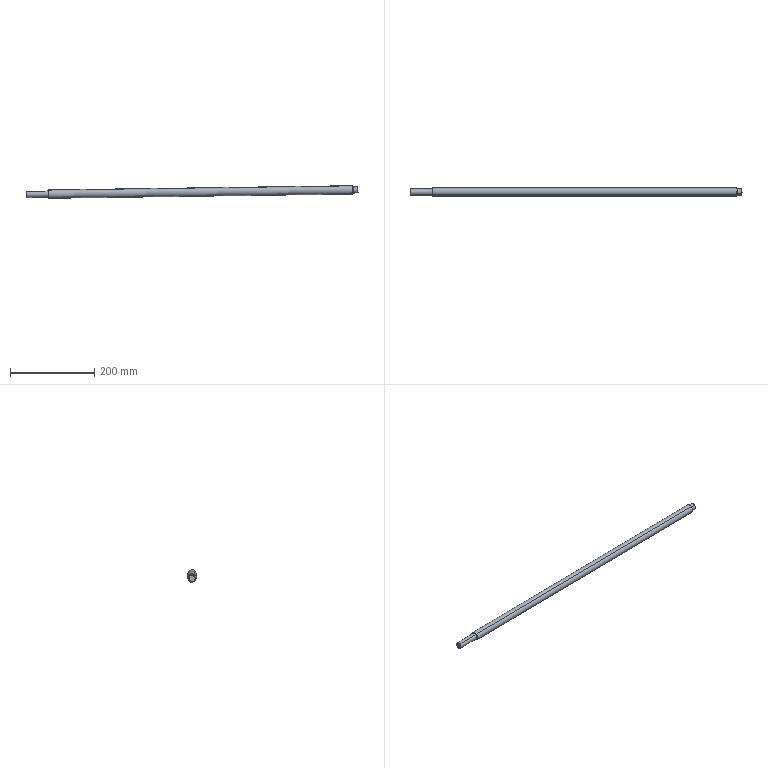Component | SolidWorks | DA-0220-Screw-4 | 1 solid | 18 faces | box 790.12 x 20.29 x 30.1 mm | volume 239115 mm3 | cylinder 6 | torus 4 | cone 4 | plane 4 | commonest cylinder face diameters 15 x4 20 x2
build123d program:
from build123d import *

# Parameters (mm, degrees)
CHAMFER1_SIZE = 0.3
FILLET1_R     = 0.5


with BuildPart() as part:
    # Sketch1 → Revolve1 (revolve)
    with BuildSketch(Plane.XY):
        Polygon((0, 7.49), (0, -0.01047), (790, -0.01047), (790, 7.49), (778, 7.49), (778, 9.99), (54, 9.99), (54, 7.49), align=None)
    revolve(axis=Axis((0, -0.01047, 0), (1, 0, 0)))

    # Chamfer1
    chamfer1_edges = [part.edges().sort_by_distance(p)[0] for p in [
        (0, -7.51, 0),
        (790, -7.51, 0),
    ]]
    chamfer(chamfer1_edges, length=CHAMFER1_SIZE)

    # Fillet1
    fillet1_edges = [part.edges().sort_by_distance(p)[0] for p in [
        (54, -7.51, 0),
        (778, -7.51, 0),
    ]]
    fillet(fillet1_edges, radius=FILLET1_R)


solid = part.part

# Placed as in the assembly
solid = solid.moved(Location((248.156, -93.945, 6.971), (44.973, -0.5493, 0.5815)))
STEP:
#1=COLOUR_RGB('',0.7922,0.8196,0.9333);
#2=FILL_AREA_STYLE_COLOUR('',#1);
#3=FILL_AREA_STYLE('',(#2));
#4=SURFACE_STYLE_FILL_AREA(#3);
#5=SURFACE_SIDE_STYLE('',(#4));
#6=SURFACE_STYLE_USAGE(.BOTH.,#5);
#7=PRESENTATION_STYLE_ASSIGNMENT((#6));
#8=CARTESIAN_POINT('',(40.413,-3.838,0.955));
#9=VERTEX_POINT('',#8);
#10=CARTESIAN_POINT('',(40.42,-3.535,0.4487));
#11=VERTEX_POINT('',#10);
#12=CARTESIAN_POINT('',(40.417,-3.687,0.7019));
#13=DIRECTION('',(0.9999,0.000404,0.01395));
#14=DIRECTION('',(0.01176,0.5145,-0.8574));
#15=AXIS2_PLACEMENT_3D('',#12,#13,#14);
#16=CIRCLE('',#15,0.2953);
#17=EDGE_CURVE('',#9,#11,#16,.T.);
#18=ORIENTED_EDGE('',*,*,#17,.F.);
#19=CARTESIAN_POINT('',(40.393,-3.849,0.9716));
#20=VERTEX_POINT('',#19);
#21=CARTESIAN_POINT('',(40.413,-3.849,0.9719));
#22=DIRECTION('',(-0.007525,0.8575,0.5144));
#23=DIRECTION('',(0.,-0.5144,0.8575));
#24=AXIS2_PLACEMENT_3D('',#21,#22,#23);
#25=CIRCLE('',#24,0.01969);
#26=EDGE_CURVE('',#9,#20,#25,.T.);
#27=ORIENTED_EDGE('',*,*,#26,.T.);
#28=CARTESIAN_POINT('',(40.401,-3.524,0.4315));
#29=VERTEX_POINT('',#28);
#30=CARTESIAN_POINT('',(40.397,-3.687,0.7016));
#31=DIRECTION('',(-0.9999,-0.000404,-0.01395));
#32=DIRECTION('',(0.01176,0.5145,-0.8574));
#33=AXIS2_PLACEMENT_3D('',#30,#31,#32);
#34=CIRCLE('',#33,0.315);
#35=EDGE_CURVE('',#29,#20,#34,.T.);
#36=ORIENTED_EDGE('',*,*,#35,.F.);
#37=CARTESIAN_POINT('',(40.42,-3.524,0.4318));
#38=DIRECTION('',(0.007525,-0.8575,-0.5144));
#39=DIRECTION('',(0.,0.5144,-0.8575));
#40=AXIS2_PLACEMENT_3D('',#37,#38,#39);
#41=CIRCLE('',#40,0.01969);
#42=EDGE_CURVE('',#11,#29,#41,.T.);
#43=ORIENTED_EDGE('',*,*,#42,.F.);
#44=EDGE_LOOP('',(#18,#27,#36,#43));
#45=FACE_OUTER_BOUND('',#44,.T.);
#46=CARTESIAN_POINT('',(40.417,-3.687,0.7019));
#47=DIRECTION('',(0.9999,0.000404,0.01395));
#48=DIRECTION('',(0.01176,0.5145,-0.8574));
#49=AXIS2_PLACEMENT_3D('',#46,#47,#48);
#50=TOROIDAL_SURFACE('',#49,0.315,0.01969);
#51=ADVANCED_FACE('',(#45),#50,.F.);
#52=CARTESIAN_POINT('',(11.879,-3.546,0.05038));
#53=VERTEX_POINT('',#52);
#54=CARTESIAN_POINT('',(11.873,-3.85,0.5567));
#55=VERTEX_POINT('',#54);
#56=CARTESIAN_POINT('',(11.876,-3.698,0.3036));
#57=DIRECTION('',(-0.9999,-0.000404,-0.01395));
#58=DIRECTION('',(-0.01176,-0.5145,0.8574));
#59=AXIS2_PLACEMENT_3D('',#56,#57,#58);
#60=CIRCLE('',#59,0.2953);
#61=EDGE_CURVE('',#53,#55,#60,.T.);
#62=ORIENTED_EDGE('',*,*,#61,.F.);
#63=CARTESIAN_POINT('',(11.899,-3.536,0.03378));
#64=VERTEX_POINT('',#63);
#65=CARTESIAN_POINT('',(11.88,-3.536,0.0335));
#66=DIRECTION('',(-0.007525,0.8575,0.5144));
#67=DIRECTION('',(0.,-0.5144,0.8575));
#68=AXIS2_PLACEMENT_3D('',#65,#66,#67);
#69=CIRCLE('',#68,0.01969);
#70=EDGE_CURVE('',#53,#64,#69,.T.);
#71=ORIENTED_EDGE('',*,*,#70,.T.);
#72=CARTESIAN_POINT('',(11.892,-3.86,0.5739));
#73=VERTEX_POINT('',#72);
#74=CARTESIAN_POINT('',(11.896,-3.698,0.3038));
#75=DIRECTION('',(0.9999,0.000404,0.01395));
#76=DIRECTION('',(-0.01176,-0.5145,0.8574));
#77=AXIS2_PLACEMENT_3D('',#74,#75,#76);
#78=CIRCLE('',#77,0.315);
#79=EDGE_CURVE('',#73,#64,#78,.T.);
#80=ORIENTED_EDGE('',*,*,#79,.F.);
#81=CARTESIAN_POINT('',(11.872,-3.86,0.5736));
#82=DIRECTION('',(0.007525,-0.8575,-0.5144));
#83=DIRECTION('',(0.,0.5144,-0.8575));
#84=AXIS2_PLACEMENT_3D('',#81,#82,#83);
#85=CIRCLE('',#84,0.01969);
#86=EDGE_CURVE('',#55,#73,#85,.T.);
#87=ORIENTED_EDGE('',*,*,#86,.F.);
#88=EDGE_LOOP('',(#62,#71,#80,#87));
#89=FACE_OUTER_BOUND('',#88,.T.);
#90=CARTESIAN_POINT('',(11.876,-3.698,0.3036));
#91=DIRECTION('',(-0.9999,-0.000404,-0.01395));
#92=DIRECTION('',(-0.01176,-0.5145,0.8574));
#93=AXIS2_PLACEMENT_3D('',#90,#91,#92);
#94=TOROIDAL_SURFACE('',#93,0.315,0.01969);
#95=ADVANCED_FACE('',(#89),#94,.F.);
#96=CARTESIAN_POINT('',(40.871,-3.929,0.5624));
#97=VERTEX_POINT('',#96);
#98=CARTESIAN_POINT('',(40.867,-3.443,0.854));
#99=VERTEX_POINT('',#98);
#100=CARTESIAN_POINT('',(40.869,-3.686,0.7082));
#101=DIRECTION('',(0.9999,0.000404,0.01395));
#102=DIRECTION('',(0.01176,0.5145,-0.8574));
#103=AXIS2_PLACEMENT_3D('',#100,#101,#102);
#104=CIRCLE('',#103,0.2835);
#105=EDGE_CURVE('',#97,#99,#104,.T.);
#106=ORIENTED_EDGE('',*,*,#105,.F.);
#107=CARTESIAN_POINT('',(40.86,-3.94,0.5561));
#108=VERTEX_POINT('',#107);
#109=CARTESIAN_POINT('',(40.871,-3.929,0.5624));
#110=DIRECTION('',(-0.7017,-0.6066,-0.3736));
#111=VECTOR('',#110,39.37);
#112=LINE('',#109,#111);
#113=EDGE_CURVE('',#97,#108,#112,.T.);
#114=ORIENTED_EDGE('',*,*,#113,.T.);
#115=CARTESIAN_POINT('',(40.861,-3.534,0.4548));
#116=VERTEX_POINT('',#115);
#117=CARTESIAN_POINT('',(40.857,-3.686,0.708));
#118=DIRECTION('',(-0.9999,-0.000404,-0.01395));
#119=DIRECTION('',(0.007525,-0.8575,-0.5144));
#120=AXIS2_PLACEMENT_3D('',#117,#118,#119);
#121=CIRCLE('',#120,0.2953);
#122=EDGE_CURVE('',#116,#108,#121,.T.);
#123=ORIENTED_EDGE('',*,*,#122,.F.);
#124=CARTESIAN_POINT('',(40.855,-3.433,0.8599));
#125=VERTEX_POINT('',#124);
#126=CARTESIAN_POINT('',(40.857,-3.686,0.708));
#127=DIRECTION('',(-0.9999,-0.000404,-0.01395));
#128=DIRECTION('',(0.007525,-0.8575,-0.5144));
#129=AXIS2_PLACEMENT_3D('',#126,#127,#128);
#130=CIRCLE('',#129,0.2953);
#131=EDGE_CURVE('',#125,#116,#130,.T.);
#132=ORIENTED_EDGE('',*,*,#131,.F.);
#133=CARTESIAN_POINT('',(40.867,-3.443,0.854));
#134=DIRECTION('',(-0.7124,0.6061,0.3539));
#135=VECTOR('',#134,39.37);
#136=LINE('',#133,#135);
#137=EDGE_CURVE('',#99,#125,#136,.T.);
#138=ORIENTED_EDGE('',*,*,#137,.F.);
#139=EDGE_LOOP('',(#106,#114,#123,#132,#138));
#140=FACE_OUTER_BOUND('',#139,.T.);
#141=CARTESIAN_POINT('',(40.869,-3.686,0.7082));
#142=DIRECTION('',(-0.9999,-0.000404,-0.01395));
#143=DIRECTION('',(-0.007525,0.8575,0.5144));
#144=AXIS2_PLACEMENT_3D('',#141,#142,#143);
#145=CONICAL_SURFACE('',#144,0.2835,0.7854);
#146=ADVANCED_FACE('',(#140),#145,.T.);
#147=CARTESIAN_POINT('',(9.768,-3.456,0.42));
#148=VERTEX_POINT('',#147);
#149=CARTESIAN_POINT('',(9.772,-3.942,0.1283));
#150=VERTEX_POINT('',#149);
#151=CARTESIAN_POINT('',(9.77,-3.699,0.2742));
#152=DIRECTION('',(-0.9999,-0.000404,-0.01395));
#153=DIRECTION('',(-0.01176,-0.5145,0.8574));
#154=AXIS2_PLACEMENT_3D('',#151,#152,#153);
#155=CIRCLE('',#154,0.2835);
#156=EDGE_CURVE('',#148,#150,#155,.T.);
#157=ORIENTED_EDGE('',*,*,#156,.F.);
#158=CARTESIAN_POINT('',(9.78,-3.446,0.4262));
#159=VERTEX_POINT('',#158);
#160=CARTESIAN_POINT('',(9.78,-3.446,0.4262));
#161=DIRECTION('',(0.7017,0.6066,0.3736));
#162=VECTOR('',#161,39.37);
#163=LINE('',#160,#162);
#164=EDGE_CURVE('',#148,#159,#163,.T.);
#165=ORIENTED_EDGE('',*,*,#164,.T.);
#166=CARTESIAN_POINT('',(9.785,-3.547,0.02115));
#167=VERTEX_POINT('',#166);
#168=CARTESIAN_POINT('',(9.782,-3.699,0.2743));
#169=DIRECTION('',(0.9999,0.000404,0.01395));
#170=DIRECTION('',(-0.007525,0.8575,0.5144));
#171=AXIS2_PLACEMENT_3D('',#168,#169,#170);
#172=CIRCLE('',#171,0.2953);
#173=EDGE_CURVE('',#167,#159,#172,.T.);
#174=ORIENTED_EDGE('',*,*,#173,.F.);
#175=CARTESIAN_POINT('',(9.784,-3.952,0.1224));
#176=VERTEX_POINT('',#175);
#177=CARTESIAN_POINT('',(9.782,-3.699,0.2743));
#178=DIRECTION('',(0.9999,0.000404,0.01395));
#179=DIRECTION('',(-0.007525,0.8575,0.5144));
#180=AXIS2_PLACEMENT_3D('',#177,#178,#179);
#181=CIRCLE('',#180,0.2953);
#182=EDGE_CURVE('',#176,#167,#181,.T.);
#183=ORIENTED_EDGE('',*,*,#182,.F.);
#184=CARTESIAN_POINT('',(9.784,-3.952,0.1224));
#185=DIRECTION('',(0.7124,-0.6061,-0.3539));
#186=VECTOR('',#185,39.37);
#187=LINE('',#184,#186);
#188=EDGE_CURVE('',#150,#176,#187,.T.);
#189=ORIENTED_EDGE('',*,*,#188,.F.);
#190=EDGE_LOOP('',(#157,#165,#174,#183,#189));
#191=FACE_OUTER_BOUND('',#190,.T.);
#192=CARTESIAN_POINT('',(9.782,-3.699,0.2743));
#193=DIRECTION('',(0.9999,0.000404,0.01395));
#194=DIRECTION('',(0.007525,-0.8575,-0.5144));
#195=AXIS2_PLACEMENT_3D('',#192,#193,#194);
#196=CONICAL_SURFACE('',#195,0.2953,0.7854);
#197=ADVANCED_FACE('',(#191),#196,.T.);
#198=ORIENTED_EDGE('',*,*,#173,.T.);
#199=CARTESIAN_POINT('',(9.778,-3.851,0.5275));
#200=VERTEX_POINT('',#199);
#201=CARTESIAN_POINT('',(9.782,-3.699,0.2743));
#202=DIRECTION('',(0.9999,0.000404,0.01395));
#203=DIRECTION('',(-0.007525,0.8575,0.5144));
#204=AXIS2_PLACEMENT_3D('',#201,#202,#203);
#205=CIRCLE('',#204,0.2953);
#206=EDGE_CURVE('',#159,#200,#205,.T.);
#207=ORIENTED_EDGE('',*,*,#206,.T.);
#208=CARTESIAN_POINT('',(9.766,-3.851,0.5273));
#209=DIRECTION('',(0.9999,0.000404,0.01395));
#210=VECTOR('',#209,39.37);
#211=LINE('',#208,#210);
#212=EDGE_CURVE('',#200,#55,#211,.T.);
#213=ORIENTED_EDGE('',*,*,#212,.T.);
#214=CARTESIAN_POINT('',(11.876,-3.698,0.3036));
#215=DIRECTION('',(-0.9999,-0.000404,-0.01395));
#216=DIRECTION('',(-0.01176,-0.5145,0.8574));
#217=AXIS2_PLACEMENT_3D('',#214,#215,#216);
#218=CIRCLE('',#217,0.2953);
#219=EDGE_CURVE('',#55,#53,#218,.T.);
#220=ORIENTED_EDGE('',*,*,#219,.T.);
#221=CARTESIAN_POINT('',(9.773,-3.547,0.02099));
#222=DIRECTION('',(0.9999,0.000404,0.01395));
#223=VECTOR('',#222,39.37);
#224=LINE('',#221,#223);
#225=EDGE_CURVE('',#167,#53,#224,.T.);
#226=ORIENTED_EDGE('',*,*,#225,.F.);
#227=EDGE_LOOP('',(#198,#207,#213,#220,#226));
#228=FACE_OUTER_BOUND('',#227,.T.);
#229=CARTESIAN_POINT('',(9.77,-3.699,0.2742));
#230=DIRECTION('',(0.9999,0.000404,0.01395));
#231=DIRECTION('',(0.01176,0.5145,-0.8574));
#232=AXIS2_PLACEMENT_3D('',#229,#230,#231);
#233=CYLINDRICAL_SURFACE('',#232,0.2953);
#234=ADVANCED_FACE('',(#228),#233,.T.);
#235=CARTESIAN_POINT('',(11.9,-3.495,-0.03374));
#236=VERTEX_POINT('',#235);
#237=CARTESIAN_POINT('',(11.891,-3.901,0.6414));
#238=VERTEX_POINT('',#237);
#239=CARTESIAN_POINT('',(11.896,-3.698,0.3038));
#240=DIRECTION('',(0.9999,0.000404,0.01395));
#241=DIRECTION('',(0.01176,0.5145,-0.8574));
#242=AXIS2_PLACEMENT_3D('',#239,#240,#241);
#243=CIRCLE('',#242,0.3937);
#244=EDGE_CURVE('',#236,#238,#243,.T.);
#245=ORIENTED_EDGE('',*,*,#244,.T.);
#246=CARTESIAN_POINT('',(40.392,-3.889,1.039));
#247=VERTEX_POINT('',#246);
#248=CARTESIAN_POINT('',(9.765,-3.901,0.6117));
#249=DIRECTION('',(0.9999,0.000404,0.01395));
#250=VECTOR('',#249,39.37);
#251=LINE('',#248,#250);
#252=EDGE_CURVE('',#238,#247,#251,.T.);
#253=ORIENTED_EDGE('',*,*,#252,.T.);
#254=CARTESIAN_POINT('',(40.401,-3.484,0.364));
#255=VERTEX_POINT('',#254);
#256=CARTESIAN_POINT('',(40.397,-3.687,0.7016));
#257=DIRECTION('',(0.9999,0.000404,0.01395));
#258=DIRECTION('',(0.01176,0.5145,-0.8574));
#259=AXIS2_PLACEMENT_3D('',#256,#257,#258);
#260=CIRCLE('',#259,0.3937);
#261=EDGE_CURVE('',#255,#247,#260,.T.);
#262=ORIENTED_EDGE('',*,*,#261,.F.);
#263=CARTESIAN_POINT('',(9.775,-3.496,-0.0634));
#264=DIRECTION('',(0.9999,0.000404,0.01395));
#265=VECTOR('',#264,39.37);
#266=LINE('',#263,#265);
#267=EDGE_CURVE('',#236,#255,#266,.T.);
#268=ORIENTED_EDGE('',*,*,#267,.F.);
#269=EDGE_LOOP('',(#245,#253,#262,#268));
#270=FACE_OUTER_BOUND('',#269,.T.);
#271=CARTESIAN_POINT('',(9.77,-3.699,0.2742));
#272=DIRECTION('',(0.9999,0.000404,0.01395));
#273=DIRECTION('',(0.01176,0.5145,-0.8574));
#274=AXIS2_PLACEMENT_3D('',#271,#272,#273);
#275=CYLINDRICAL_SURFACE('',#274,0.3937);
#276=ADVANCED_FACE('',(#270),#275,.T.);
#277=CARTESIAN_POINT('',(40.417,-3.687,0.7019));
#278=DIRECTION('',(0.9999,0.000404,0.01395));
#279=DIRECTION('',(0.01176,0.5145,-0.8574));
#280=AXIS2_PLACEMENT_3D('',#277,#278,#279);
#281=CIRCLE('',#280,0.2953);
#282=EDGE_CURVE('',#11,#9,#281,.T.);
#283=ORIENTED_EDGE('',*,*,#282,.T.);
#284=CARTESIAN_POINT('',(40.854,-3.838,0.9612));
#285=VERTEX_POINT('',#284);
#286=CARTESIAN_POINT('',(9.766,-3.851,0.5273));
#287=DIRECTION('',(0.9999,0.000404,0.01395));
#288=VECTOR('',#287,39.37);
#289=LINE('',#286,#288);
#290=EDGE_CURVE('',#9,#285,#289,.T.);
#291=ORIENTED_EDGE('',*,*,#290,.T.);
#292=CARTESIAN_POINT('',(40.857,-3.686,0.708));
#293=DIRECTION('',(-0.9999,-0.000404,-0.01395));
#294=DIRECTION('',(0.007525,-0.8575,-0.5144));
#295=AXIS2_PLACEMENT_3D('',#292,#293,#294);
#296=CIRCLE('',#295,0.2953);
#297=EDGE_CURVE('',#285,#125,#296,.T.);
#298=ORIENTED_EDGE('',*,*,#297,.T.);
#299=ORIENTED_EDGE('',*,*,#131,.T.);
#300=CARTESIAN_POINT('',(9.773,-3.547,0.02099));
#301=DIRECTION('',(0.9999,0.000404,0.01395));
#302=VECTOR('',#301,39.37);
#303=LINE('',#300,#302);
#304=EDGE_CURVE('',#11,#116,#303,.T.);
#305=ORIENTED_EDGE('',*,*,#304,.F.);
#306=EDGE_LOOP('',(#283,#291,#298,#299,#305));
#307=FACE_OUTER_BOUND('',#306,.T.);
#308=CARTESIAN_POINT('',(9.77,-3.699,0.2742));
#309=DIRECTION('',(0.9999,0.000404,0.01395));
#310=DIRECTION('',(0.01176,0.5145,-0.8574));
#311=AXIS2_PLACEMENT_3D('',#308,#309,#310);
#312=CYLINDRICAL_SURFACE('',#311,0.2953);
#313=ADVANCED_FACE('',(#307),#312,.T.);
#314=CARTESIAN_POINT('',(40.869,-3.686,0.7082));
#315=DIRECTION('',(0.9999,0.000404,0.01395));
#316=DIRECTION('',(0.01176,0.5145,-0.8574));
#317=AXIS2_PLACEMENT_3D('',#314,#315,#316);
#318=CIRCLE('',#317,0.2835);
#319=EDGE_CURVE('',#99,#97,#318,.T.);
#320=ORIENTED_EDGE('',*,*,#319,.T.);
#321=ORIENTED_EDGE('',*,*,#105,.T.);
#322=EDGE_LOOP('',(#320,#321));
#323=FACE_OUTER_BOUND('',#322,.T.);
#324=CARTESIAN_POINT('',(40.869,-3.686,0.7082));
#325=DIRECTION('',(0.9999,0.000404,0.01395));
#326=DIRECTION('',(0.01176,0.5145,-0.8574));
#327=AXIS2_PLACEMENT_3D('',#324,#325,#326);
#328=PLANE('',#327);
#329=ADVANCED_FACE('',(#323),#328,.T.);
#330=ORIENTED_EDGE('',*,*,#290,.F.);
#331=ORIENTED_EDGE('',*,*,#17,.T.);
#332=ORIENTED_EDGE('',*,*,#304,.T.);
#333=ORIENTED_EDGE('',*,*,#122,.T.);
#334=CARTESIAN_POINT('',(40.857,-3.686,0.708));
#335=DIRECTION('',(-0.9999,-0.000404,-0.01395));
#336=DIRECTION('',(0.007525,-0.8575,-0.5144));
#337=AXIS2_PLACEMENT_3D('',#334,#335,#336);
#338=CIRCLE('',#337,0.2953);
#339=EDGE_CURVE('',#108,#285,#338,.T.);
#340=ORIENTED_EDGE('',*,*,#339,.T.);
#341=EDGE_LOOP('',(#330,#331,#332,#333,#340));
#342=FACE_OUTER_BOUND('',#341,.T.);
#343=CARTESIAN_POINT('',(9.77,-3.699,0.2742));
#344=DIRECTION('',(0.9999,0.000404,0.01395));
#345=DIRECTION('',(0.01176,0.5145,-0.8574));
#346=AXIS2_PLACEMENT_3D('',#343,#344,#345);
#347=CYLINDRICAL_SURFACE('',#346,0.2953);
#348=ADVANCED_FACE('',(#342),#347,.T.);
#349=ORIENTED_EDGE('',*,*,#35,.T.);
#350=CARTESIAN_POINT('',(40.397,-3.687,0.7016));
#351=DIRECTION('',(-0.9999,-0.000404,-0.01395));
#352=DIRECTION('',(0.01176,0.5145,-0.8574));
#353=AXIS2_PLACEMENT_3D('',#350,#351,#352);
#354=CIRCLE('',#353,0.315);
#355=EDGE_CURVE('',#20,#29,#354,.T.);
#356=ORIENTED_EDGE('',*,*,#355,.T.);
#357=EDGE_LOOP('',(#349,#356));
#358=FACE_BOUND('',#357,.T.);
#359=ORIENTED_EDGE('',*,*,#261,.T.);
#360=CARTESIAN_POINT('',(40.397,-3.687,0.7016));
#361=DIRECTION('',(0.9999,0.000404,0.01395));
#362=DIRECTION('',(0.01176,0.5145,-0.8574));
#363=AXIS2_PLACEMENT_3D('',#360,#361,#362);
#364=CIRCLE('',#363,0.3937);
#365=EDGE_CURVE('',#247,#255,#364,.T.);
#366=ORIENTED_EDGE('',*,*,#365,.T.);
#367=EDGE_LOOP('',(#359,#366));
#368=FACE_OUTER_BOUND('',#367,.T.);
#369=CARTESIAN_POINT('',(40.4,-3.535,0.4484));
#370=DIRECTION('',(0.9999,0.000404,0.01395));
#371=DIRECTION('',(0.01176,0.5145,-0.8574));
#372=AXIS2_PLACEMENT_3D('',#369,#370,#371);
#373=PLANE('',#372);
#374=ADVANCED_FACE('',(#358,#368),#373,.T.);
#375=ORIENTED_EDGE('',*,*,#252,.F.);
#376=CARTESIAN_POINT('',(11.896,-3.698,0.3038));
#377=DIRECTION('',(0.9999,0.000404,0.01395));
#378=DIRECTION('',(0.01176,0.5145,-0.8574));
#379=AXIS2_PLACEMENT_3D('',#376,#377,#378);
#380=CIRCLE('',#379,0.3937);
#381=EDGE_CURVE('',#238,#236,#380,.T.);
#382=ORIENTED_EDGE('',*,*,#381,.T.);
#383=ORIENTED_EDGE('',*,*,#267,.T.);
#384=ORIENTED_EDGE('',*,*,#365,.F.);
#385=EDGE_LOOP('',(#375,#382,#383,#384));
#386=FACE_OUTER_BOUND('',#385,.T.);
#387=CARTESIAN_POINT('',(9.77,-3.699,0.2742));
#388=DIRECTION('',(0.9999,0.000404,0.01395));
#389=DIRECTION('',(0.01176,0.5145,-0.8574));
#390=AXIS2_PLACEMENT_3D('',#387,#388,#389);
#391=CYLINDRICAL_SURFACE('',#390,0.3937);
#392=ADVANCED_FACE('',(#386),#391,.T.);
#393=ORIENTED_EDGE('',*,*,#79,.T.);
#394=CARTESIAN_POINT('',(11.896,-3.698,0.3038));
#395=DIRECTION('',(0.9999,0.000404,0.01395));
#396=DIRECTION('',(-0.01176,-0.5145,0.8574));
#397=AXIS2_PLACEMENT_3D('',#394,#395,#396);
#398=CIRCLE('',#397,0.315);
#399=EDGE_CURVE('',#64,#73,#398,.T.);
#400=ORIENTED_EDGE('',*,*,#399,.T.);
#401=EDGE_LOOP('',(#393,#400));
#402=FACE_BOUND('',#401,.T.);
#403=ORIENTED_EDGE('',*,*,#244,.F.);
#404=ORIENTED_EDGE('',*,*,#381,.F.);
#405=EDGE_LOOP('',(#403,#404));
#406=FACE_OUTER_BOUND('',#405,.T.);
#407=CARTESIAN_POINT('',(11.9,-3.495,-0.03374));
#408=DIRECTION('',(-0.9999,-0.000404,-0.01395));
#409=DIRECTION('',(-0.01176,-0.5145,0.8574));
#410=AXIS2_PLACEMENT_3D('',#407,#408,#409);
#411=PLANE('',#410);
#412=ADVANCED_FACE('',(#402,#406),#411,.T.);
#413=ORIENTED_EDGE('',*,*,#212,.F.);
#414=CARTESIAN_POINT('',(9.782,-3.699,0.2743));
#415=DIRECTION('',(0.9999,0.000404,0.01395));
#416=DIRECTION('',(-0.007525,0.8575,0.5144));
#417=AXIS2_PLACEMENT_3D('',#414,#415,#416);
#418=CIRCLE('',#417,0.2953);
#419=EDGE_CURVE('',#200,#176,#418,.T.);
#420=ORIENTED_EDGE('',*,*,#419,.T.);
#421=ORIENTED_EDGE('',*,*,#182,.T.);
#422=ORIENTED_EDGE('',*,*,#225,.T.);
#423=ORIENTED_EDGE('',*,*,#61,.T.);
#424=EDGE_LOOP('',(#413,#420,#421,#422,#423));
#425=FACE_OUTER_BOUND('',#424,.T.);
#426=CARTESIAN_POINT('',(9.77,-3.699,0.2742));
#427=DIRECTION('',(0.9999,0.000404,0.01395));
#428=DIRECTION('',(0.01176,0.5145,-0.8574));
#429=AXIS2_PLACEMENT_3D('',#426,#427,#428);
#430=CYLINDRICAL_SURFACE('',#429,0.2953);
#431=ADVANCED_FACE('',(#425),#430,.T.);
#432=CARTESIAN_POINT('',(9.77,-3.699,0.2742));
#433=DIRECTION('',(-0.9999,-0.000404,-0.01395));
#434=DIRECTION('',(-0.01176,-0.5145,0.8574));
#435=AXIS2_PLACEMENT_3D('',#432,#433,#434);
#436=CIRCLE('',#435,0.2835);
#437=EDGE_CURVE('',#150,#148,#436,.T.);
#438=ORIENTED_EDGE('',*,*,#437,.T.);
#439=ORIENTED_EDGE('',*,*,#156,.T.);
#440=EDGE_LOOP('',(#438,#439));
#441=FACE_OUTER_BOUND('',#440,.T.);
#442=CARTESIAN_POINT('',(9.773,-3.547,0.02099));
#443=DIRECTION('',(-0.9999,-0.000404,-0.01395));
#444=DIRECTION('',(-0.01176,-0.5145,0.8574));
#445=AXIS2_PLACEMENT_3D('',#442,#443,#444);
#446=PLANE('',#445);
#447=ADVANCED_FACE('',(#441),#446,.T.);
#448=ORIENTED_EDGE('',*,*,#164,.F.);
#449=ORIENTED_EDGE('',*,*,#437,.F.);
#450=ORIENTED_EDGE('',*,*,#188,.T.);
#451=ORIENTED_EDGE('',*,*,#419,.F.);
#452=ORIENTED_EDGE('',*,*,#206,.F.);
#453=EDGE_LOOP('',(#448,#449,#450,#451,#452));
#454=FACE_OUTER_BOUND('',#453,.T.);
#455=CARTESIAN_POINT('',(9.782,-3.699,0.2743));
#456=DIRECTION('',(0.9999,0.000404,0.01395));
#457=DIRECTION('',(0.007525,-0.8575,-0.5144));
#458=AXIS2_PLACEMENT_3D('',#455,#456,#457);
#459=CONICAL_SURFACE('',#458,0.2953,0.7854);
#460=ADVANCED_FACE('',(#454),#459,.T.);
#461=ORIENTED_EDGE('',*,*,#113,.F.);
#462=ORIENTED_EDGE('',*,*,#319,.F.);
#463=ORIENTED_EDGE('',*,*,#137,.T.);
#464=ORIENTED_EDGE('',*,*,#297,.F.);
#465=ORIENTED_EDGE('',*,*,#339,.F.);
#466=EDGE_LOOP('',(#461,#462,#463,#464,#465));
#467=FACE_OUTER_BOUND('',#466,.T.);
#468=CARTESIAN_POINT('',(40.869,-3.686,0.7082));
#469=DIRECTION('',(-0.9999,-0.000404,-0.01395));
#470=DIRECTION('',(-0.007525,0.8575,0.5144));
#471=AXIS2_PLACEMENT_3D('',#468,#469,#470);
#472=CONICAL_SURFACE('',#471,0.2835,0.7854);
#473=ADVANCED_FACE('',(#467),#472,.T.);
#474=ORIENTED_EDGE('',*,*,#70,.F.);
#475=ORIENTED_EDGE('',*,*,#219,.F.);
#476=ORIENTED_EDGE('',*,*,#86,.T.);
#477=ORIENTED_EDGE('',*,*,#399,.F.);
#478=EDGE_LOOP('',(#474,#475,#476,#477));
#479=FACE_OUTER_BOUND('',#478,.T.);
#480=CARTESIAN_POINT('',(11.876,-3.698,0.3036));
#481=DIRECTION('',(-0.9999,-0.000404,-0.01395));
#482=DIRECTION('',(-0.01176,-0.5145,0.8574));
#483=AXIS2_PLACEMENT_3D('',#480,#481,#482);
#484=TOROIDAL_SURFACE('',#483,0.315,0.01969);
#485=ADVANCED_FACE('',(#479),#484,.F.);
#486=ORIENTED_EDGE('',*,*,#26,.F.);
#487=ORIENTED_EDGE('',*,*,#282,.F.);
#488=ORIENTED_EDGE('',*,*,#42,.T.);
#489=ORIENTED_EDGE('',*,*,#355,.F.);
#490=EDGE_LOOP('',(#486,#487,#488,#489));
#491=FACE_OUTER_BOUND('',#490,.T.);
#492=CARTESIAN_POINT('',(40.417,-3.687,0.7019));
#493=DIRECTION('',(0.9999,0.000404,0.01395));
#494=DIRECTION('',(0.01176,0.5145,-0.8574));
#495=AXIS2_PLACEMENT_3D('',#492,#493,#494);
#496=TOROIDAL_SURFACE('',#495,0.315,0.01969);
#497=ADVANCED_FACE('',(#491),#496,.F.);
#498=CLOSED_SHELL('',(#51,#95,#146,#197,#234,#276,#313,#329,#348,#374,#392,#412,#431,#447,#460,#473,#485,#497));
#499=MANIFOLD_SOLID_BREP('',#498);
#500=STYLED_ITEM('',(#7),#499);
#501=(LENGTH_UNIT()NAMED_UNIT(*)SI_UNIT($,.METRE.));
#502=LENGTH_MEASURE_WITH_UNIT(LENGTH_MEASURE(0.0254),#501);
#503=DIMENSIONAL_EXPONENTS(1.,0.,0.,0.,0.,0.,0.);
#504=(CONVERSION_BASED_UNIT('',#502)LENGTH_UNIT()NAMED_UNIT(#503));
#505=UNCERTAINTY_MEASURE_WITH_UNIT(LENGTH_MEASURE(0.00001),#504,'','');
#506=(NAMED_UNIT(*)PLANE_ANGLE_UNIT()SI_UNIT($,.RADIAN.));
#507=(NAMED_UNIT(*)SI_UNIT($,.STERADIAN.)SOLID_ANGLE_UNIT());
#508=(GEOMETRIC_REPRESENTATION_CONTEXT(3)GLOBAL_UNCERTAINTY_ASSIGNED_CONTEXT((#505))GLOBAL_UNIT_ASSIGNED_CONTEXT((#504,#506,#507))REPRESENTATION_CONTEXT('',''));
#509=MECHANICAL_DESIGN_GEOMETRIC_PRESENTATION_REPRESENTATION('',(#500),#508);
#510=PRESENTATION_LAYER_ASSIGNMENT('','',(#500));
#511=CARTESIAN_POINT('',(0.,0.,0.));
#512=DIRECTION('',(0.,0.,1.));
#513=DIRECTION('',(1.,0.,0.));
#514=AXIS2_PLACEMENT_3D('',#511,#512,#513);
#515=(LENGTH_UNIT()NAMED_UNIT(*)SI_UNIT($,.METRE.));
#516=LENGTH_MEASURE_WITH_UNIT(LENGTH_MEASURE(0.0254),#515);
#517=DIMENSIONAL_EXPONENTS(1.,0.,0.,0.,0.,0.,0.);
#518=(CONVERSION_BASED_UNIT('',#516)LENGTH_UNIT()NAMED_UNIT(#517));
#519=UNCERTAINTY_MEASURE_WITH_UNIT(LENGTH_MEASURE(0.00001),#518,'','');
#520=(NAMED_UNIT(*)PLANE_ANGLE_UNIT()SI_UNIT($,.RADIAN.));
#521=(NAMED_UNIT(*)SI_UNIT($,.STERADIAN.)SOLID_ANGLE_UNIT());
#522=(GEOMETRIC_REPRESENTATION_CONTEXT(3)GLOBAL_UNCERTAINTY_ASSIGNED_CONTEXT((#519))GLOBAL_UNIT_ASSIGNED_CONTEXT((#518,#520,#521))REPRESENTATION_CONTEXT('',''));
#523=ADVANCED_BREP_SHAPE_REPRESENTATION('',(#499,#514),#522);